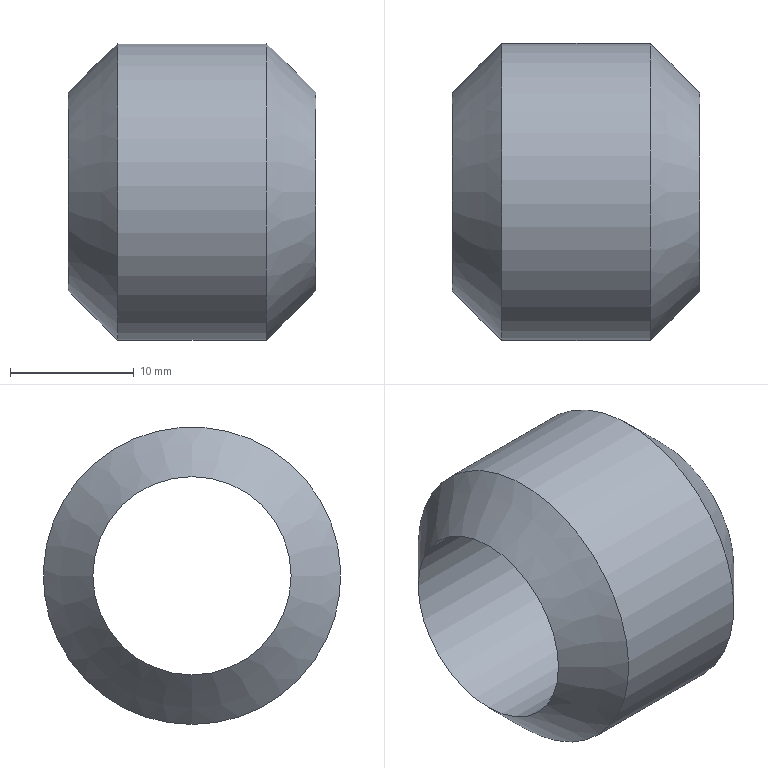Component | NX | PACKING | 1 solid | 4 faces | box 20 x 24 x 24 mm | volume 3954 mm3 | cylinder 2 | cone 2 | commonest cylinder face diameters 24 x1 16 x1
STEP:
#1=CARTESIAN_POINT('',(0.,0.,0.));
#2=DIRECTION('',(0.,0.,1.));
#3=DIRECTION('',(1.,0.,0.));
#4=AXIS2_PLACEMENT_3D('',#1,#2,#3);
#5=CARTESIAN_POINT('',(7.795,0.,-12.));
#6=VERTEX_POINT('',#5);
#7=CARTESIAN_POINT('',(7.795,0.,0.));
#8=DIRECTION('',(1.,0.,0.));
#9=DIRECTION('',(0.,0.,-1.));
#10=AXIS2_PLACEMENT_3D('',#7,#8,#9);
#11=CIRCLE('',#10,12.);
#12=CARTESIAN_POINT('',(23.795,0.,0.));
#13=DIRECTION('',(-1.,0.,0.));
#14=DIRECTION('',(0.,0.,1.));
#15=AXIS2_PLACEMENT_3D('',#12,#13,#14);
#16=CYLINDRICAL_SURFACE('',#15,12.);
#17=CARTESIAN_POINT('',(9.425,16.));
#18=DIRECTION('',(-1.,0.));
#19=VECTOR('',#18,1.);
#20=LINE('',#17,#19);
#21=(GEOMETRIC_REPRESENTATION_CONTEXT(2)PARAMETRIC_REPRESENTATION_CONTEXT()REPRESENTATION_CONTEXT('',''));
#22=DEFINITIONAL_REPRESENTATION('',(#20),#21);
#23=PCURVE('',#16,#22);
#24=CARTESIAN_POINT('',(7.795,0.,0.));
#25=DIRECTION('',(1.,0.,0.));
#26=DIRECTION('',(0.,0.,-1.));
#27=AXIS2_PLACEMENT_3D('',#24,#25,#26);
#28=CONICAL_SURFACE('',#27,12.,0.7854);
#29=CARTESIAN_POINT('',(0.,0.));
#30=DIRECTION('',(1.,0.));
#31=VECTOR('',#30,1.);
#32=LINE('',#29,#31);
#33=(GEOMETRIC_REPRESENTATION_CONTEXT(2)PARAMETRIC_REPRESENTATION_CONTEXT()REPRESENTATION_CONTEXT('',''));
#34=DEFINITIONAL_REPRESENTATION('',(#32),#33);
#35=PCURVE('',#28,#34);
#36=SURFACE_CURVE('',#11,(#23,#35),.PCURVE_S1.);
#37=EDGE_CURVE('',#6,#6,#36,.T.);
#38=ORIENTED_EDGE('',*,*,#37,.T.);
#39=CARTESIAN_POINT('',(19.795,0.,-12.));
#40=VERTEX_POINT('',#39);
#41=CARTESIAN_POINT('',(19.795,0.,-12.));
#42=CARTESIAN_POINT('',(7.795,0.,-12.));
#43=B_SPLINE_CURVE_WITH_KNOTS('',1,(#41,#42),.UNSPECIFIED.,.F.,.F.,(2,2),(4.,16.),.PIECEWISE_BEZIER_KNOTS.);
#44=CARTESIAN_POINT('',(3.142,0.));
#45=DIRECTION('',(0.,1.));
#46=VECTOR('',#45,1.);
#47=LINE('',#44,#46);
#48=(GEOMETRIC_REPRESENTATION_CONTEXT(2)PARAMETRIC_REPRESENTATION_CONTEXT()REPRESENTATION_CONTEXT('',''));
#49=DEFINITIONAL_REPRESENTATION('',(#47),#48);
#50=PCURVE('',#16,#49);
#51=CARTESIAN_POINT('',(9.425,0.));
#52=DIRECTION('',(0.,1.));
#53=VECTOR('',#52,1.);
#54=LINE('',#51,#53);
#55=(GEOMETRIC_REPRESENTATION_CONTEXT(2)PARAMETRIC_REPRESENTATION_CONTEXT()REPRESENTATION_CONTEXT('',''));
#56=DEFINITIONAL_REPRESENTATION('',(#54),#55);
#57=PCURVE('',#16,#56);
#58=SEAM_CURVE('',#43,(#50,#57),.PCURVE_S1.);
#59=EDGE_CURVE('',#40,#6,#58,.T.);
#60=ORIENTED_EDGE('',*,*,#59,.F.);
#61=CARTESIAN_POINT('',(19.795,0.,0.));
#62=DIRECTION('',(-1.,0.,0.));
#63=DIRECTION('',(0.,0.,-1.));
#64=AXIS2_PLACEMENT_3D('',#61,#62,#63);
#65=CIRCLE('',#64,12.);
#66=CARTESIAN_POINT('',(3.142,4.));
#67=DIRECTION('',(1.,0.));
#68=VECTOR('',#67,1.);
#69=LINE('',#66,#68);
#70=(GEOMETRIC_REPRESENTATION_CONTEXT(2)PARAMETRIC_REPRESENTATION_CONTEXT()REPRESENTATION_CONTEXT('',''));
#71=DEFINITIONAL_REPRESENTATION('',(#69),#70);
#72=PCURVE('',#16,#71);
#73=CARTESIAN_POINT('',(23.795,0.,0.));
#74=DIRECTION('',(-1.,0.,0.));
#75=DIRECTION('',(0.,0.,1.));
#76=AXIS2_PLACEMENT_3D('',#73,#74,#75);
#77=CONICAL_SURFACE('',#76,8.,0.7854);
#78=CARTESIAN_POINT('',(3.142,4.));
#79=DIRECTION('',(1.,0.));
#80=VECTOR('',#79,1.);
#81=LINE('',#78,#80);
#82=(GEOMETRIC_REPRESENTATION_CONTEXT(2)PARAMETRIC_REPRESENTATION_CONTEXT()REPRESENTATION_CONTEXT('',''));
#83=DEFINITIONAL_REPRESENTATION('',(#81),#82);
#84=PCURVE('',#77,#83);
#85=SURFACE_CURVE('',#65,(#72,#84),.PCURVE_S1.);
#86=EDGE_CURVE('',#40,#40,#85,.T.);
#87=ORIENTED_EDGE('',*,*,#86,.T.);
#88=ORIENTED_EDGE('',*,*,#59,.T.);
#89=EDGE_LOOP('',(#38,#60,#87,#88));
#90=FACE_BOUND('',#89,.T.);
#91=ADVANCED_FACE('',(#90),#16,.T.);
#92=CARTESIAN_POINT('',(23.795,0.,-8.));
#93=VERTEX_POINT('',#92);
#94=CARTESIAN_POINT('',(23.795,0.,0.));
#95=DIRECTION('',(1.,0.,0.));
#96=DIRECTION('',(0.,0.,-1.));
#97=AXIS2_PLACEMENT_3D('',#94,#95,#96);
#98=CIRCLE('',#97,8.);
#99=CARTESIAN_POINT('',(23.795,0.,0.));
#100=DIRECTION('',(-1.,0.,0.));
#101=DIRECTION('',(0.,0.,1.));
#102=AXIS2_PLACEMENT_3D('',#99,#100,#101);
#103=CYLINDRICAL_SURFACE('',#102,8.);
#104=CARTESIAN_POINT('',(9.425,0.));
#105=DIRECTION('',(-1.,0.));
#106=VECTOR('',#105,1.);
#107=LINE('',#104,#106);
#108=(GEOMETRIC_REPRESENTATION_CONTEXT(2)PARAMETRIC_REPRESENTATION_CONTEXT()REPRESENTATION_CONTEXT('',''));
#109=DEFINITIONAL_REPRESENTATION('',(#107),#108);
#110=PCURVE('',#103,#109);
#111=CARTESIAN_POINT('',(9.425,0.));
#112=DIRECTION('',(-1.,0.));
#113=VECTOR('',#112,1.);
#114=LINE('',#111,#113);
#115=(GEOMETRIC_REPRESENTATION_CONTEXT(2)PARAMETRIC_REPRESENTATION_CONTEXT()REPRESENTATION_CONTEXT('',''));
#116=DEFINITIONAL_REPRESENTATION('',(#114),#115);
#117=PCURVE('',#77,#116);
#118=SURFACE_CURVE('',#98,(#110,#117),.PCURVE_S1.);
#119=EDGE_CURVE('',#93,#93,#118,.T.);
#120=ORIENTED_EDGE('',*,*,#119,.F.);
#121=CARTESIAN_POINT('',(3.795,0.,-8.));
#122=VERTEX_POINT('',#121);
#123=CARTESIAN_POINT('',(23.795,0.,-8.));
#124=CARTESIAN_POINT('',(3.795,0.,-8.));
#125=B_SPLINE_CURVE_WITH_KNOTS('',1,(#123,#124),.UNSPECIFIED.,.F.,.F.,(2,2),(0.,20.),.PIECEWISE_BEZIER_KNOTS.);
#126=CARTESIAN_POINT('',(9.425,0.));
#127=DIRECTION('',(0.,1.));
#128=VECTOR('',#127,1.);
#129=LINE('',#126,#128);
#130=(GEOMETRIC_REPRESENTATION_CONTEXT(2)PARAMETRIC_REPRESENTATION_CONTEXT()REPRESENTATION_CONTEXT('',''));
#131=DEFINITIONAL_REPRESENTATION('',(#129),#130);
#132=PCURVE('',#103,#131);
#133=CARTESIAN_POINT('',(3.142,0.));
#134=DIRECTION('',(0.,1.));
#135=VECTOR('',#134,1.);
#136=LINE('',#133,#135);
#137=(GEOMETRIC_REPRESENTATION_CONTEXT(2)PARAMETRIC_REPRESENTATION_CONTEXT()REPRESENTATION_CONTEXT('',''));
#138=DEFINITIONAL_REPRESENTATION('',(#136),#137);
#139=PCURVE('',#103,#138);
#140=SEAM_CURVE('',#125,(#132,#139),.PCURVE_S1.);
#141=EDGE_CURVE('',#93,#122,#140,.T.);
#142=ORIENTED_EDGE('',*,*,#141,.T.);
#143=CARTESIAN_POINT('',(3.795,0.,0.));
#144=DIRECTION('',(1.,0.,0.));
#145=DIRECTION('',(0.,0.,-1.));
#146=AXIS2_PLACEMENT_3D('',#143,#144,#145);
#147=CIRCLE('',#146,8.);
#148=CARTESIAN_POINT('',(9.425,20.));
#149=DIRECTION('',(-1.,0.));
#150=VECTOR('',#149,1.);
#151=LINE('',#148,#150);
#152=(GEOMETRIC_REPRESENTATION_CONTEXT(2)PARAMETRIC_REPRESENTATION_CONTEXT()REPRESENTATION_CONTEXT('',''));
#153=DEFINITIONAL_REPRESENTATION('',(#151),#152);
#154=PCURVE('',#103,#153);
#155=CARTESIAN_POINT('',(0.,-4.));
#156=DIRECTION('',(1.,0.));
#157=VECTOR('',#156,1.);
#158=LINE('',#155,#157);
#159=(GEOMETRIC_REPRESENTATION_CONTEXT(2)PARAMETRIC_REPRESENTATION_CONTEXT()REPRESENTATION_CONTEXT('',''));
#160=DEFINITIONAL_REPRESENTATION('',(#158),#159);
#161=PCURVE('',#28,#160);
#162=SURFACE_CURVE('',#147,(#154,#161),.PCURVE_S1.);
#163=EDGE_CURVE('',#122,#122,#162,.T.);
#164=ORIENTED_EDGE('',*,*,#163,.T.);
#165=ORIENTED_EDGE('',*,*,#141,.F.);
#166=EDGE_LOOP('',(#120,#142,#164,#165));
#167=FACE_BOUND('',#166,.F.);
#168=ADVANCED_FACE('',(#167),#103,.F.);
#169=ORIENTED_EDGE('',*,*,#163,.T.);
#170=CARTESIAN_POINT('',(3.795,0.,-8.));
#171=CARTESIAN_POINT('',(7.795,0.,-12.));
#172=B_SPLINE_CURVE_WITH_KNOTS('',1,(#170,#171),.UNSPECIFIED.,.F.,.F.,(2,2),(-5.657,0.),.PIECEWISE_BEZIER_KNOTS.);
#173=CARTESIAN_POINT('',(6.283,0.));
#174=DIRECTION('',(0.,1.));
#175=VECTOR('',#174,1.);
#176=LINE('',#173,#175);
#177=(GEOMETRIC_REPRESENTATION_CONTEXT(2)PARAMETRIC_REPRESENTATION_CONTEXT()REPRESENTATION_CONTEXT('',''));
#178=DEFINITIONAL_REPRESENTATION('',(#176),#177);
#179=PCURVE('',#28,#178);
#180=CARTESIAN_POINT('',(0.,0.));
#181=DIRECTION('',(0.,1.));
#182=VECTOR('',#181,1.);
#183=LINE('',#180,#182);
#184=(GEOMETRIC_REPRESENTATION_CONTEXT(2)PARAMETRIC_REPRESENTATION_CONTEXT()REPRESENTATION_CONTEXT('',''));
#185=DEFINITIONAL_REPRESENTATION('',(#183),#184);
#186=PCURVE('',#28,#185);
#187=SEAM_CURVE('',#172,(#179,#186),.PCURVE_S1.);
#188=EDGE_CURVE('',#122,#6,#187,.T.);
#189=ORIENTED_EDGE('',*,*,#188,.T.);
#190=ORIENTED_EDGE('',*,*,#37,.F.);
#191=ORIENTED_EDGE('',*,*,#188,.F.);
#192=EDGE_LOOP('',(#169,#189,#190,#191));
#193=FACE_BOUND('',#192,.T.);
#194=ADVANCED_FACE('',(#193),#28,.T.);
#195=ORIENTED_EDGE('',*,*,#86,.F.);
#196=CARTESIAN_POINT('',(23.795,0.,-8.));
#197=CARTESIAN_POINT('',(19.795,0.,-12.));
#198=B_SPLINE_CURVE_WITH_KNOTS('',1,(#196,#197),.UNSPECIFIED.,.F.,.F.,(2,2),(0.,5.657),.PIECEWISE_BEZIER_KNOTS.);
#199=CARTESIAN_POINT('',(3.142,0.));
#200=DIRECTION('',(0.,1.));
#201=VECTOR('',#200,1.);
#202=LINE('',#199,#201);
#203=(GEOMETRIC_REPRESENTATION_CONTEXT(2)PARAMETRIC_REPRESENTATION_CONTEXT()REPRESENTATION_CONTEXT('',''));
#204=DEFINITIONAL_REPRESENTATION('',(#202),#203);
#205=PCURVE('',#77,#204);
#206=CARTESIAN_POINT('',(9.425,0.));
#207=DIRECTION('',(0.,1.));
#208=VECTOR('',#207,1.);
#209=LINE('',#206,#208);
#210=(GEOMETRIC_REPRESENTATION_CONTEXT(2)PARAMETRIC_REPRESENTATION_CONTEXT()REPRESENTATION_CONTEXT('',''));
#211=DEFINITIONAL_REPRESENTATION('',(#209),#210);
#212=PCURVE('',#77,#211);
#213=SEAM_CURVE('',#198,(#205,#212),.PCURVE_S1.);
#214=EDGE_CURVE('',#93,#40,#213,.T.);
#215=ORIENTED_EDGE('',*,*,#214,.F.);
#216=ORIENTED_EDGE('',*,*,#119,.F.);
#217=ORIENTED_EDGE('',*,*,#214,.T.);
#218=EDGE_LOOP('',(#195,#215,#216,#217));
#219=FACE_BOUND('',#218,.T.);
#220=ADVANCED_FACE('',(#219),#77,.T.);
#221=CLOSED_SHELL('',(#91,#168,#194,#220));
#222=MANIFOLD_SOLID_BREP('',#221);
#223=(LENGTH_UNIT()NAMED_UNIT(*)SI_UNIT(.MILLI.,.METRE.));
#224=UNCERTAINTY_MEASURE_WITH_UNIT(LENGTH_MEASURE(0.00001),#223,'','');
#225=(NAMED_UNIT(*)PLANE_ANGLE_UNIT()SI_UNIT($,.RADIAN.));
#226=(NAMED_UNIT(*)SI_UNIT($,.STERADIAN.)SOLID_ANGLE_UNIT());
#227=(GEOMETRIC_REPRESENTATION_CONTEXT(3)GLOBAL_UNCERTAINTY_ASSIGNED_CONTEXT((#224))GLOBAL_UNIT_ASSIGNED_CONTEXT((#223,#225,#226))REPRESENTATION_CONTEXT('',''));
#228=ADVANCED_BREP_SHAPE_REPRESENTATION('',(#4,#222),#227);